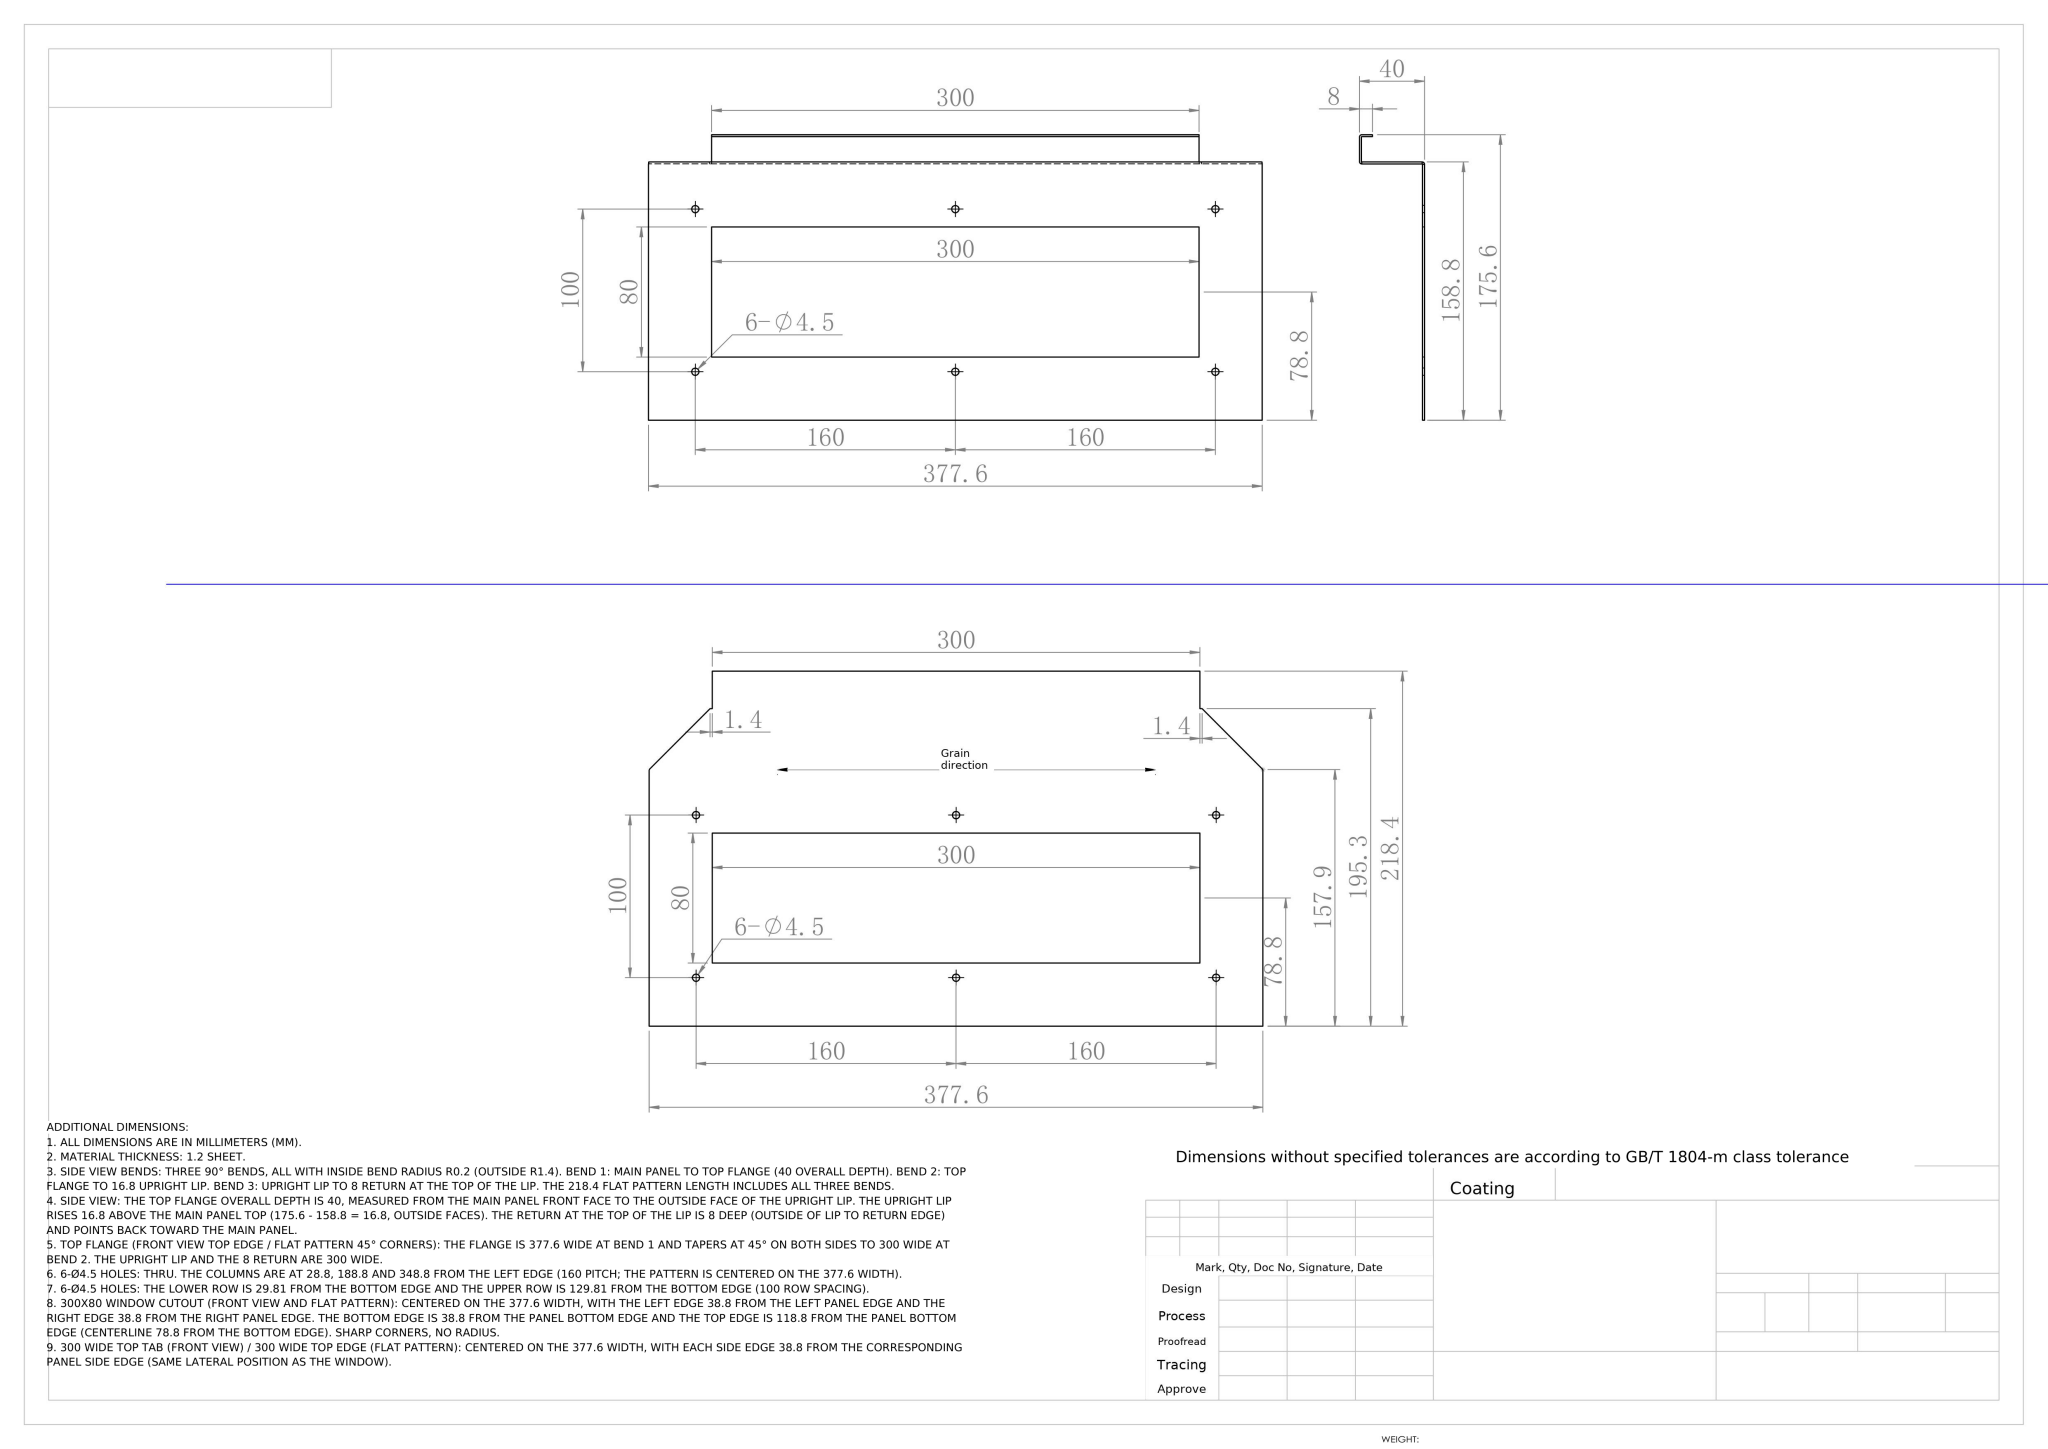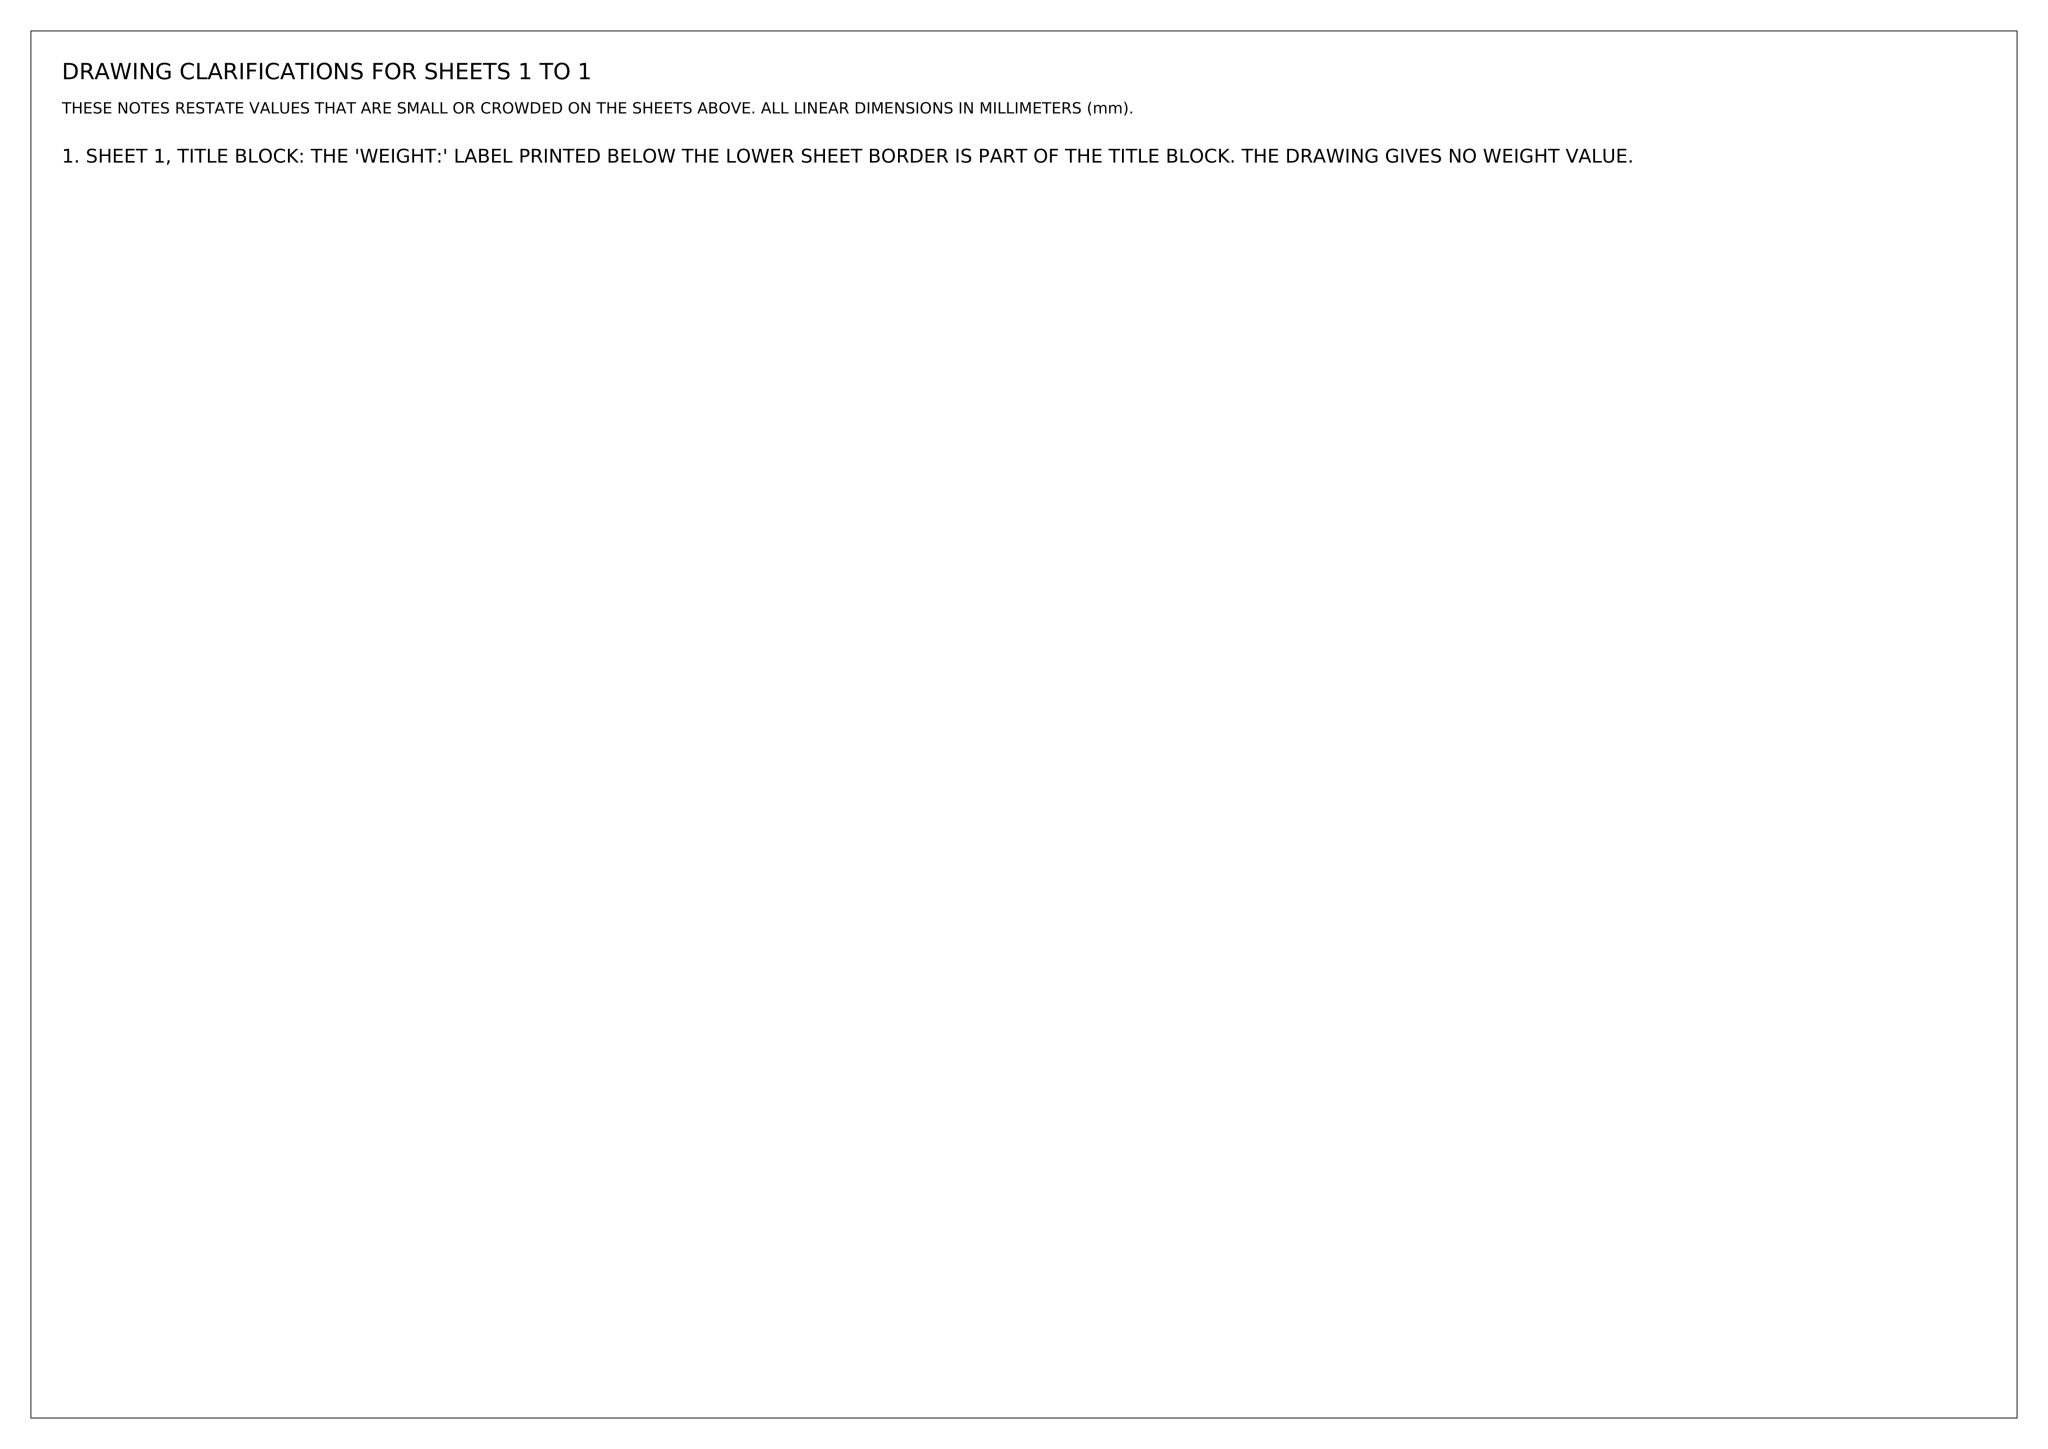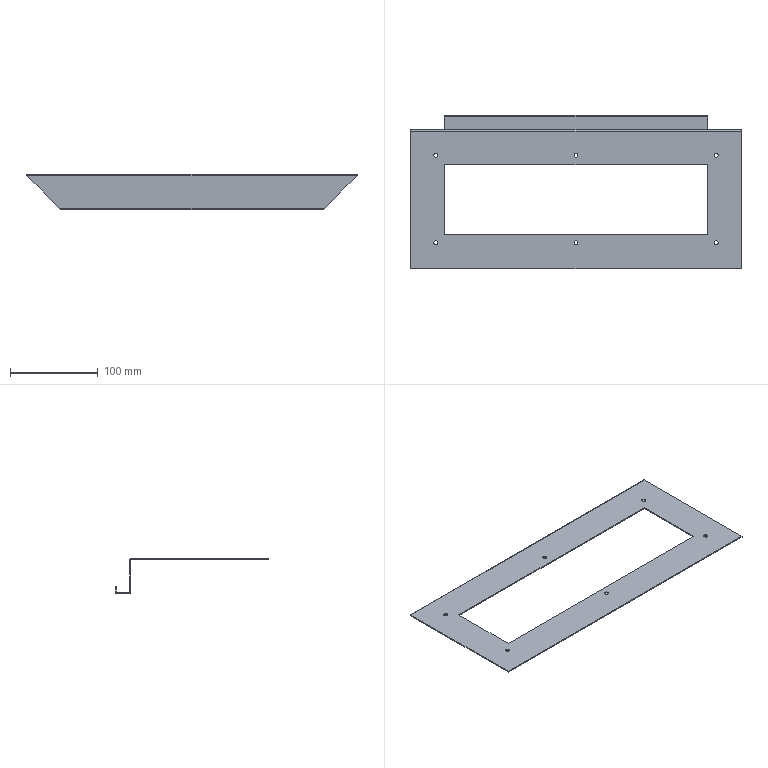Part | NX | mm | 1 solid | 48 faces | box 377.6 x 175.6 x 40 mm | volume 66906 mm3 | plane 28 | cylinder 18 | spline 2 | commonest cylinder face diameters 4.5 x12 2.8 x3 0.4 x3